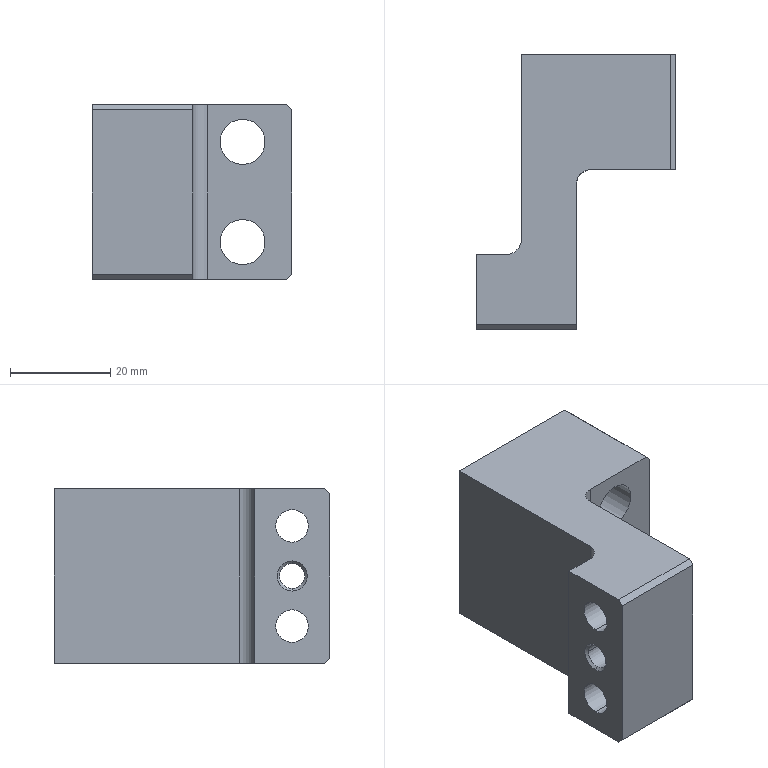Component | SolidWorks | ChainPartSupport-2 | 1 solid | 36 faces | box 39.8 x 55 x 34.8 mm | volume 36175 mm3 | cylinder 16 | plane 16 | cone 4 | commonest cylinder face diameters 11 x4 6.5 x4 9 x4 5 x2 6 x2
build123d program:
from build123d import *

# Parameters (mm, degrees)
BOSS_EXTRUDE1_DEPTH                                  = 17.4
F_9_0_9_DIAMETER_HOLE1_D                             = 9
HOLE_SIZE_ACCORDING_TO_THE_TYPE_OF_HEX_S_D           = 6.5
HOLE_SIZE_ACCORDING_TO_THE_TYPE_OF_HEX_S_CBORE_D     = 11
HOLE_SIZE_ACCORDING_TO_THE_TYPE_OF_HEX_S_CBORE_DEPTH = 7
CHAMFER1_SIZE                                        = 1
FILLET2_R                                            = 3
SKETCH9_W                                            = 34.8
SKETCH9_H                                            = 40
CUT_EXTRUDE1_DEPTH                                   = 9
FILLET3_R                                            = 3
SKETCH10_R                                           = 2.5
CUT_EXTRUDE2_DEPTH                                   = 62.055
CHAMFER2_SIZE                                        = 0.5


with BuildPart() as part:
    # Sketch1 → Boss-Extrude1 (new, symmetric)
    with BuildSketch(Plane.XY):
        Polygon((0, 0), (-20, 0), (-20, -55), (19.8, -55), (19.8, -32), (0, -32), align=None)
    extrude(amount=BOSS_EXTRUDE1_DEPTH, both=True)

    # 9.0 _9_ Diameter Hole1 (through all)
    with Locations(Plane(origin=(0, -32, 0), x_dir=(-1, 0, 0), z_dir=(0, 1, 0))):
        with Locations((-10, -10), (-10, 10)):
            Hole(F_9_0_9_DIAMETER_HOLE1_D / 2)

    # Hole Size according to the type of Hex S (through all)
    with Locations(Plane(origin=(0, 0, 0), x_dir=(0, 0, -1), z_dir=(1, 0, 0))):
        with Locations((-10, -7.5), (10, -7.5)):
            CounterBoreHole(HOLE_SIZE_ACCORDING_TO_THE_TYPE_OF_HEX_S_D / 2, HOLE_SIZE_ACCORDING_TO_THE_TYPE_OF_HEX_S_CBORE_D / 2, HOLE_SIZE_ACCORDING_TO_THE_TYPE_OF_HEX_S_CBORE_DEPTH)

    # Chamfer1
    chamfer1_edges = [part.edges().sort_by_distance(p)[0] for p in [
        (19.8, -43.5, 17.4),
        (19.8, -43.5, -17.4),
        (-10, 0, 17.4),
        (-10, 0, -17.4),
    ]]
    chamfer(chamfer1_edges, length=CHAMFER1_SIZE)

    # Fillet2
    fillet2_edges = [part.edges().sort_by_distance(p)[0] for p in [
        (0, -32, 0),
    ]]
    fillet(fillet2_edges, radius=FILLET2_R)

    # Sketch9 → Cut-Extrude1 (cut)
    with BuildSketch(Plane.ZY.offset(20)):
        with Locations((0, -35)):
            Rectangle(SKETCH9_W, SKETCH9_H)
    extrude(amount=-CUT_EXTRUDE1_DEPTH, mode=Mode.SUBTRACT)

    # Fillet3
    fillet3_edges = [part.edges().sort_by_distance(p)[0] for p in [
        (-11, -15, 0),
    ]]
    fillet(fillet3_edges, radius=FILLET3_R)

    # Sketch10 → Cut-Extrude2 (cut, through all)
    with BuildSketch(Plane(origin=(0, 0, 0), x_dir=(0, 0, -1), z_dir=(1, 0, 0))):
        with Locations(Location((0, -7.5, 0), (0, 0, 90))):
            Circle(SKETCH10_R)
    extrude(amount=-CUT_EXTRUDE2_DEPTH, mode=Mode.SUBTRACT)

    # Chamfer2
    chamfer2_edges = [part.edges().sort_by_distance(p)[0] for p in [
        (-20, -10, 0),
        (0, -10, 0),
    ]]
    chamfer(chamfer2_edges, length=CHAMFER2_SIZE)


solid = part.part

# Placed as in the assembly
solid = solid.moved(Location((155.637, 19.937, -590.304), (180, 0, 0)))